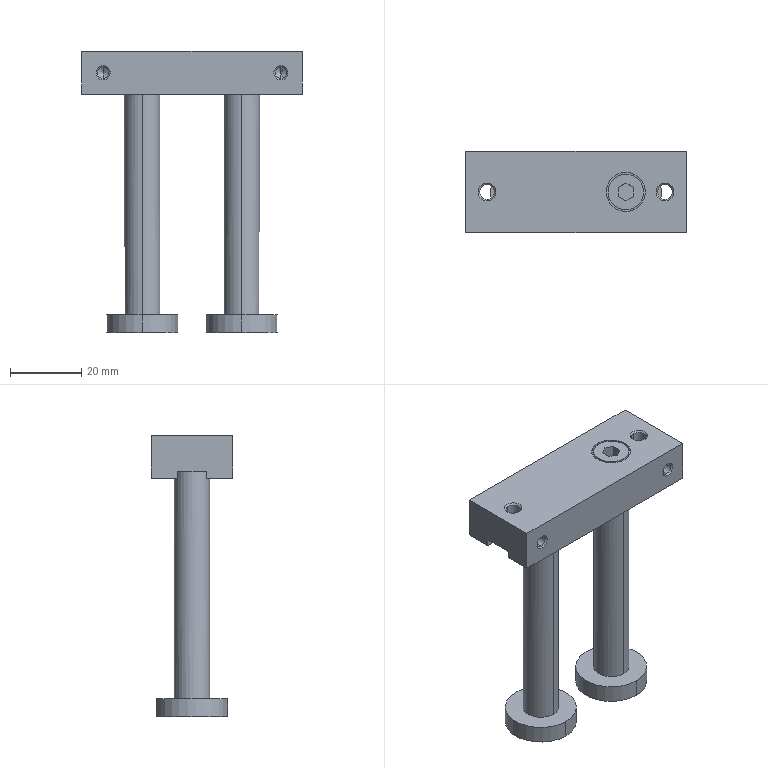Component | SolidWorks | CXSM20-20-Z73(0_0_0)-1_CXSM20-20(0_0)_ROD-1 | 1 solid | 90 faces | box 62 x 23 x 79 mm | volume 28643 mm3 | plane 38 | cylinder 28 | cone 24 | commonest cylinder face diameters 3.242 x8 10 x6 4.134 x4 20 x4 7 x2 8 x2 11 x2
build123d program:
from build123d import *

# Parameters (mm, degrees)
SKETCH1_W           = 23
SKETCH1_H           = 62
BOSS_EXTRUDE1_DEPTH = 12
SKETCH2_W           = 8
SKETCH2_H           = 62
CUT_EXTRUDE1_DEPTH  = 2
CUT_EXTRUDE2_START  = -1
SKETCH11_R          = 5.5
SKETCH11_R_2        = 5
CUT_EXTRUDE2_DEPTH  = 1
CUT_EXTRUDE3_DEPTH  = 4.33
SKETCH13_R          = 4
SKETCH13_R_2        = 3.5
CUT_EXTRUDE4_DEPTH  = 1
CUT_EXTRUDE5_DEPTH  = 4


with BuildPart() as part:
    # Sketch1 → Boss-Extrude1 (new body)
    with BuildSketch(Plane.XY.offset(12)):
        Rectangle(SKETCH1_W, SKETCH1_H)
    extrude(amount=BOSS_EXTRUDE1_DEPTH)

    # Sketch2 → Cut-Extrude1 (cut)
    with BuildSketch(Plane.XY.offset(12)):
        Rectangle(SKETCH2_W, SKETCH2_H)
    extrude(amount=CUT_EXTRUDE1_DEPTH, mode=Mode.SUBTRACT)

    # Sketch3 → Revolve1 (revolve)
    with BuildSketch(Plane(origin=(0, 0, 0), x_dir=(0, 0, -1), z_dir=(1, 0, 0)), mode=Mode.PRIVATE) as revolve1_sk:
        Polygon((-17, 14), (-17, 19), (50, 19), (50, 24), (55, 24), (55, 14), align=None)
    revolve(revolve1_sk.sketch.rotate(Axis((0, 14, -55), (0, 0, 1)), 270), axis=Axis((0, 14, -55), (0, 0, 1)))

    # Sketch4 → Revolve2 (revolve)
    with BuildSketch(Plane(origin=(0, 0, 0), x_dir=(0, 0, -1), z_dir=(1, 0, 0)), mode=Mode.PRIVATE) as revolve2_sk:
        Polygon((-17, -14), (-17, -9), (50, -9), (50, -4), (55, -4), (55, -14), align=None)
    revolve(revolve2_sk.sketch.rotate(Axis((0, -14, -55), (0, 0, 1)), 270), axis=Axis((0, -14, -55), (0, 0, 1)))

    # Sketch5 → Cut-Revolve1 (revolve, cut)
    with BuildSketch(Plane(origin=(0, 0, 0), x_dir=(0, 0, -1), z_dir=(1, 0, 0)), mode=Mode.PRIVATE) as cut_revolve1_sk:
        Polygon((-24, 25), (-24, 27.5), (-23.567, 27.067), (-14.433, 27.067), (-14, 27.5), (-14, 25), align=None)
    revolve(cut_revolve1_sk.sketch.rotate(Axis((0, 25, 14), (0, 0, 1)), 270), axis=Axis((0, 25, 14), (0, 0, 1)), mode=Mode.SUBTRACT)

    # Sketch6 → Cut-Revolve2 (revolve, cut)
    with BuildSketch(Plane(origin=(0, 0, 0), x_dir=(0, 0, -1), z_dir=(1, 0, 0)), mode=Mode.PRIVATE) as cut_revolve2_sk:
        Polygon((-24, -25), (-24, -22.5), (-23.567, -22.933), (-14.433, -22.933), (-14, -22.5), (-14, -25), align=None)
    revolve(cut_revolve2_sk.sketch.rotate(Axis((0, -25, 14), (0, 0, 1)), 270), axis=Axis((0, -25, 14), (0, 0, 1)), mode=Mode.SUBTRACT)

    # Sketch7 → Cut-Revolve3 (revolve, cut)
    with BuildSketch(Plane.XY.offset(18), mode=Mode.PRIVATE) as cut_revolve3_sk:
        Polygon((-11.5, 25), (-11.5, 27), (-11.121, 26.621), (-5.5, 26.621), (-4.564, 25), align=None)
    revolve(cut_revolve3_sk.sketch.rotate(Axis((-4.564, 25, 18), (-1, 0, 0)), 270), axis=Axis((-4.564, 25, 18), (-1, 0, 0)), mode=Mode.SUBTRACT)

    # Sketch8 → Cut-Revolve4 (revolve, cut)
    with BuildSketch(Plane.XY.offset(18), mode=Mode.PRIVATE) as cut_revolve4_sk:
        Polygon((-4.564, -25), (-5.5, -26.621), (-11.121, -26.621), (-11.5, -27), (-11.5, -25), align=None)
    revolve(cut_revolve4_sk.sketch.rotate(Axis((-11.5, -25, 18), (1, 0, 0)), 90), axis=Axis((-11.5, -25, 18), (1, 0, 0)), mode=Mode.SUBTRACT)

    # Sketch9 → Cut-Revolve5 (revolve, cut)
    with BuildSketch(Plane.XY.offset(18), mode=Mode.PRIVATE) as cut_revolve5_sk:
        Polygon((4.564, 25), (5.5, 26.621), (11.121, 26.621), (11.5, 27), (11.5, 25), align=None)
    revolve(cut_revolve5_sk.sketch.rotate(Axis((11.5, 25, 18), (-1, 0, 0)), 270), axis=Axis((11.5, 25, 18), (-1, 0, 0)), mode=Mode.SUBTRACT)

    # Sketch10 → Cut-Revolve6 (revolve, cut)
    with BuildSketch(Plane.XY.offset(18), mode=Mode.PRIVATE) as cut_revolve6_sk:
        Polygon((11.5, -25), (11.5, -27), (11.121, -26.621), (5.5, -26.621), (4.564, -25), align=None)
    revolve(cut_revolve6_sk.sketch.rotate(Axis((4.564, -25, 18), (1, 0, 0)), 90), axis=Axis((4.564, -25, 18), (1, 0, 0)), mode=Mode.SUBTRACT)

    # Sketch11 → Cut-Extrude2 (cut)
    with BuildSketch(Plane.XY.offset(24).offset(CUT_EXTRUDE2_START)):
        with Locations((0, -14)):
            Circle(SKETCH11_R)
        with Locations((0, -14)):
            Circle(SKETCH11_R_2, mode=Mode.SUBTRACT)
    extrude(amount=CUT_EXTRUDE2_DEPTH, mode=Mode.SUBTRACT)

    # Sketch12 → Cut-Extrude3 (cut)
    with BuildSketch(Plane.XY.offset(24)):
        Polygon((-2.5, -14), (-1.25, -16.165), (1.25, -16.165), (2.5, -14), (1.25, -11.835), (-1.25, -11.835), align=None)
    extrude(amount=-CUT_EXTRUDE3_DEPTH, mode=Mode.SUBTRACT)

    # Sketch13 → Cut-Extrude4 (cut)
    with BuildSketch(Plane(origin=(11.5, 0, 0), x_dir=(0, 0, -1), z_dir=(1, 0, 0))):
        with Locations((-18, 14)):
            Circle(SKETCH13_R)
        with Locations((-18, 14)):
            Circle(SKETCH13_R_2, mode=Mode.SUBTRACT)
    extrude(amount=-CUT_EXTRUDE4_DEPTH, mode=Mode.SUBTRACT)

    # Sketch14 → Cut-Extrude5 (cut)
    with BuildSketch(Plane(origin=(11.5, 0, 0), x_dir=(0, 0, -1), z_dir=(1, 0, 0))):
        Polygon((-20.309, 14), (-19.155, 12), (-16.845, 12), (-15.691, 14), (-16.845, 16), (-19.155, 16), align=None)
    extrude(amount=-CUT_EXTRUDE5_DEPTH, mode=Mode.SUBTRACT)


solid = part.part

# Placed as in the assembly
solid = solid.moved(Location((955.264, 384.593, -336.196), (0, 0, 90)))